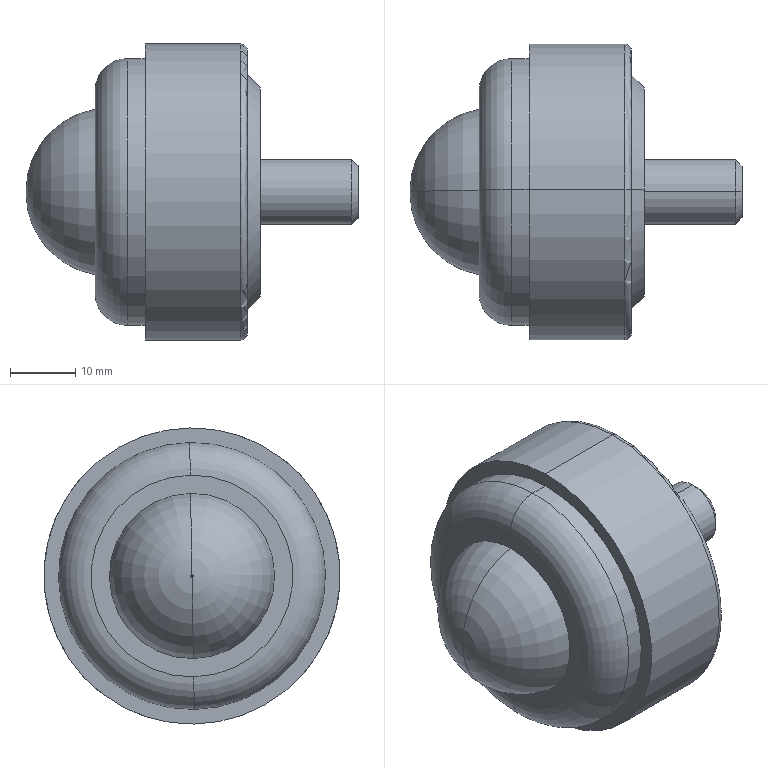Component | SolidWorks | GuideWheelAssembly-1_WD-03UniversalBall-1 | 1 solid | 22 faces | box 51 x 45.5 x 45.5 mm | volume 41338 mm3 | cylinder 6 | torus 6 | plane 6 | cone 4 | commonest cylinder face diameters 10 x2 41 x2 45.5 x2 | material Nylon 101
STEP:
#1=COLOUR_RGB('',0.7922,0.8196,0.9333);
#2=FILL_AREA_STYLE_COLOUR('',#1);
#3=FILL_AREA_STYLE('',(#2));
#4=SURFACE_STYLE_FILL_AREA(#3);
#5=SURFACE_SIDE_STYLE('',(#4));
#6=SURFACE_STYLE_USAGE(.BOTH.,#5);
#7=PRESENTATION_STYLE_ASSIGNMENT((#6));
#8=CARTESIAN_POINT('',(-21.614,-0.002693,0.8268));
#9=VERTEX_POINT('',#8);
#10=CARTESIAN_POINT('',(-21.614,0.002693,1.142));
#11=VERTEX_POINT('',#10);
#12=CARTESIAN_POINT('',(-21.614,-0.,0.9843));
#13=DIRECTION('',(1.,-0.,-0.));
#14=DIRECTION('',(0.,-0.0171,-0.9999));
#15=AXIS2_PLACEMENT_3D('',#12,#13,#14);
#16=CIRCLE('',#15,0.1575);
#17=EDGE_CURVE('',#9,#11,#16,.T.);
#18=ORIENTED_EDGE('',*,*,#17,.F.);
#19=CARTESIAN_POINT('',(-21.654,-0.003366,0.7874));
#20=VERTEX_POINT('',#19);
#21=CARTESIAN_POINT('',(-21.614,-0.002693,0.8268));
#22=DIRECTION('',(-0.7071,-0.01209,-0.707));
#23=VECTOR('',#22,39.37);
#24=LINE('',#21,#23);
#25=EDGE_CURVE('',#9,#20,#24,.T.);
#26=ORIENTED_EDGE('',*,*,#25,.T.);
#27=CARTESIAN_POINT('',(-21.654,0.003366,1.181));
#28=VERTEX_POINT('',#27);
#29=CARTESIAN_POINT('',(-21.654,-0.,0.9843));
#30=DIRECTION('',(-1.,0.,0.));
#31=DIRECTION('',(0.,-0.0171,-0.9999));
#32=AXIS2_PLACEMENT_3D('',#29,#30,#31);
#33=CIRCLE('',#32,0.1969);
#34=EDGE_CURVE('',#28,#20,#33,.T.);
#35=ORIENTED_EDGE('',*,*,#34,.F.);
#36=CARTESIAN_POINT('',(-21.614,0.002693,1.142));
#37=DIRECTION('',(-0.7071,0.01209,0.707));
#38=VECTOR('',#37,39.37);
#39=LINE('',#36,#38);
#40=EDGE_CURVE('',#11,#28,#39,.T.);
#41=ORIENTED_EDGE('',*,*,#40,.F.);
#42=EDGE_LOOP('',(#18,#26,#35,#41));
#43=FACE_OUTER_BOUND('',#42,.T.);
#44=CARTESIAN_POINT('',(-21.614,-0.,0.9843));
#45=DIRECTION('',(-1.,0.,0.));
#46=DIRECTION('',(0.,0.0171,0.9999));
#47=AXIS2_PLACEMENT_3D('',#44,#45,#46);
#48=CONICAL_SURFACE('',#47,0.1575,0.7854);
#49=ADVANCED_FACE('',(#43),#48,.T.);
#50=ORIENTED_EDGE('',*,*,#34,.T.);
#51=CARTESIAN_POINT('',(-22.205,-0.003366,0.7874));
#52=VERTEX_POINT('',#51);
#53=CARTESIAN_POINT('',(-21.614,-0.003366,0.7874));
#54=DIRECTION('',(-1.,0.,0.));
#55=VECTOR('',#54,39.37);
#56=LINE('',#53,#55);
#57=EDGE_CURVE('',#20,#52,#56,.T.);
#58=ORIENTED_EDGE('',*,*,#57,.T.);
#59=CARTESIAN_POINT('',(-22.205,0.003366,1.181));
#60=VERTEX_POINT('',#59);
#61=CARTESIAN_POINT('',(-22.205,-0.,0.9843));
#62=DIRECTION('',(1.,-0.,-0.));
#63=DIRECTION('',(0.,0.0171,0.9999));
#64=AXIS2_PLACEMENT_3D('',#61,#62,#63);
#65=CIRCLE('',#64,0.1969);
#66=EDGE_CURVE('',#52,#60,#65,.T.);
#67=ORIENTED_EDGE('',*,*,#66,.T.);
#68=CARTESIAN_POINT('',(-21.614,0.003366,1.181));
#69=DIRECTION('',(-1.,0.,0.));
#70=VECTOR('',#69,39.37);
#71=LINE('',#68,#70);
#72=EDGE_CURVE('',#28,#60,#71,.T.);
#73=ORIENTED_EDGE('',*,*,#72,.F.);
#74=EDGE_LOOP('',(#50,#58,#67,#73));
#75=FACE_OUTER_BOUND('',#74,.T.);
#76=CARTESIAN_POINT('',(-21.614,-0.,0.9843));
#77=DIRECTION('',(-1.,0.,0.));
#78=DIRECTION('',(0.,0.0171,0.9999));
#79=AXIS2_PLACEMENT_3D('',#76,#77,#78);
#80=CYLINDRICAL_SURFACE('',#79,0.1969);
#81=ADVANCED_FACE('',(#75),#80,.T.);
#82=CARTESIAN_POINT('',(-22.283,-0.01464,0.1281));
#83=VERTEX_POINT('',#82);
#84=CARTESIAN_POINT('',(-22.283,0.01464,1.84));
#85=VERTEX_POINT('',#84);
#86=CARTESIAN_POINT('',(-22.283,-0.,0.9843));
#87=DIRECTION('',(1.,-0.,-0.));
#88=DIRECTION('',(0.,0.0171,0.9999));
#89=AXIS2_PLACEMENT_3D('',#86,#87,#88);
#90=CIRCLE('',#89,0.8563);
#91=EDGE_CURVE('',#83,#85,#90,.T.);
#92=ORIENTED_EDGE('',*,*,#91,.F.);
#93=CARTESIAN_POINT('',(-22.323,-0.01532,0.08871));
#94=VERTEX_POINT('',#93);
#95=CARTESIAN_POINT('',(-22.323,-0.01464,0.1281));
#96=DIRECTION('',(0.,0.9999,-0.0171));
#97=DIRECTION('',(0.,0.0171,0.9999));
#98=AXIS2_PLACEMENT_3D('',#95,#96,#97);
#99=CIRCLE('',#98,0.03937);
#100=EDGE_CURVE('',#83,#94,#99,.T.);
#101=ORIENTED_EDGE('',*,*,#100,.T.);
#102=CARTESIAN_POINT('',(-22.323,0.01532,1.88));
#103=VERTEX_POINT('',#102);
#104=CARTESIAN_POINT('',(-22.323,-0.,0.9843));
#105=DIRECTION('',(-1.,0.,0.));
#106=DIRECTION('',(0.,0.0171,0.9999));
#107=AXIS2_PLACEMENT_3D('',#104,#105,#106);
#108=CIRCLE('',#107,0.8957);
#109=EDGE_CURVE('',#103,#94,#108,.T.);
#110=ORIENTED_EDGE('',*,*,#109,.F.);
#111=CARTESIAN_POINT('',(-22.323,0.01464,1.84));
#112=DIRECTION('',(-0.,-0.9999,0.0171));
#113=DIRECTION('',(0.,-0.0171,-0.9999));
#114=AXIS2_PLACEMENT_3D('',#111,#112,#113);
#115=CIRCLE('',#114,0.03937);
#116=EDGE_CURVE('',#85,#103,#115,.T.);
#117=ORIENTED_EDGE('',*,*,#116,.F.);
#118=EDGE_LOOP('',(#92,#101,#110,#117));
#119=FACE_OUTER_BOUND('',#118,.T.);
#120=CARTESIAN_POINT('',(-22.323,-0.,0.9843));
#121=DIRECTION('',(-1.,0.,0.));
#122=DIRECTION('',(0.,0.0171,0.9999));
#123=AXIS2_PLACEMENT_3D('',#120,#121,#122);
#124=TOROIDAL_SURFACE('',#123,0.8563,0.03937);
#125=ADVANCED_FACE('',(#119),#124,.T.);
#126=CARTESIAN_POINT('',(-22.205,-0.01077,0.3544));
#127=VERTEX_POINT('',#126);
#128=CARTESIAN_POINT('',(-22.205,0.01077,1.614));
#129=VERTEX_POINT('',#128);
#130=CARTESIAN_POINT('',(-22.205,-0.,0.9843));
#131=DIRECTION('',(1.,-0.,-0.));
#132=DIRECTION('',(0.,-0.0171,-0.9999));
#133=AXIS2_PLACEMENT_3D('',#130,#131,#132);
#134=CIRCLE('',#133,0.6299);
#135=EDGE_CURVE('',#127,#129,#134,.T.);
#136=ORIENTED_EDGE('',*,*,#135,.F.);
#137=CARTESIAN_POINT('',(-22.283,-0.01212,0.2757));
#138=VERTEX_POINT('',#137);
#139=CARTESIAN_POINT('',(-22.283,-0.01212,0.2757));
#140=DIRECTION('',(-0.7071,-0.01209,-0.707));
#141=VECTOR('',#140,39.37);
#142=LINE('',#139,#141);
#143=EDGE_CURVE('',#127,#138,#142,.T.);
#144=ORIENTED_EDGE('',*,*,#143,.T.);
#145=CARTESIAN_POINT('',(-22.283,0.01212,1.693));
#146=VERTEX_POINT('',#145);
#147=CARTESIAN_POINT('',(-22.283,-0.,0.9843));
#148=DIRECTION('',(1.,-0.,-0.));
#149=DIRECTION('',(0.,-0.0171,-0.9999));
#150=AXIS2_PLACEMENT_3D('',#147,#148,#149);
#151=CIRCLE('',#150,0.7087);
#152=EDGE_CURVE('',#138,#146,#151,.T.);
#153=ORIENTED_EDGE('',*,*,#152,.T.);
#154=CARTESIAN_POINT('',(-22.283,0.01212,1.693));
#155=DIRECTION('',(-0.7071,0.01209,0.707));
#156=VECTOR('',#155,39.37);
#157=LINE('',#154,#156);
#158=EDGE_CURVE('',#129,#146,#157,.T.);
#159=ORIENTED_EDGE('',*,*,#158,.F.);
#160=EDGE_LOOP('',(#136,#144,#153,#159));
#161=FACE_OUTER_BOUND('',#160,.T.);
#162=CARTESIAN_POINT('',(-22.283,-0.,0.9843));
#163=DIRECTION('',(-1.,0.,0.));
#164=DIRECTION('',(0.,0.0171,0.9999));
#165=AXIS2_PLACEMENT_3D('',#162,#163,#164);
#166=CONICAL_SURFACE('',#165,0.7087,0.7854);
#167=ADVANCED_FACE('',(#161),#166,.T.);
#168=CARTESIAN_POINT('',(-23.008,-0.0138,0.1773));
#169=VERTEX_POINT('',#168);
#170=CARTESIAN_POINT('',(-23.008,0.0138,1.791));
#171=VERTEX_POINT('',#170);
#172=CARTESIAN_POINT('',(-23.008,-0.,0.9843));
#173=DIRECTION('',(1.,-0.,-0.));
#174=DIRECTION('',(0.,0.0171,0.9999));
#175=AXIS2_PLACEMENT_3D('',#172,#173,#174);
#176=CIRCLE('',#175,0.8071);
#177=EDGE_CURVE('',#169,#171,#176,.T.);
#178=ORIENTED_EDGE('',*,*,#177,.F.);
#179=CARTESIAN_POINT('',(-23.205,-0.01044,0.3741));
#180=VERTEX_POINT('',#179);
#181=CARTESIAN_POINT('',(-23.008,-0.01044,0.3741));
#182=DIRECTION('',(0.,0.9999,-0.0171));
#183=DIRECTION('',(0.,0.0171,0.9999));
#184=AXIS2_PLACEMENT_3D('',#181,#182,#183);
#185=CIRCLE('',#184,0.1969);
#186=EDGE_CURVE('',#169,#180,#185,.T.);
#187=ORIENTED_EDGE('',*,*,#186,.T.);
#188=CARTESIAN_POINT('',(-23.205,0.01044,1.594));
#189=VERTEX_POINT('',#188);
#190=CARTESIAN_POINT('',(-23.205,-0.,0.9843));
#191=DIRECTION('',(-1.,0.,0.));
#192=DIRECTION('',(0.,0.0171,0.9999));
#193=AXIS2_PLACEMENT_3D('',#190,#191,#192);
#194=CIRCLE('',#193,0.6102);
#195=EDGE_CURVE('',#189,#180,#194,.T.);
#196=ORIENTED_EDGE('',*,*,#195,.F.);
#197=CARTESIAN_POINT('',(-23.008,0.01044,1.594));
#198=DIRECTION('',(-0.,-0.9999,0.0171));
#199=DIRECTION('',(0.,-0.0171,-0.9999));
#200=AXIS2_PLACEMENT_3D('',#197,#198,#199);
#201=CIRCLE('',#200,0.1969);
#202=EDGE_CURVE('',#171,#189,#201,.T.);
#203=ORIENTED_EDGE('',*,*,#202,.F.);
#204=EDGE_LOOP('',(#178,#187,#196,#203));
#205=FACE_OUTER_BOUND('',#204,.T.);
#206=CARTESIAN_POINT('',(-23.008,-0.,0.9843));
#207=DIRECTION('',(-1.,0.,0.));
#208=DIRECTION('',(0.,0.0171,0.9999));
#209=AXIS2_PLACEMENT_3D('',#206,#207,#208);
#210=TOROIDAL_SURFACE('',#209,0.6102,0.1969);
#211=ADVANCED_FACE('',(#205),#210,.T.);
#212=CARTESIAN_POINT('',(-23.622,0.0001177,0.9911));
#213=VERTEX_POINT('',#212);
#214=CARTESIAN_POINT('',(-23.622,-0.0001177,0.9774));
#215=VERTEX_POINT('',#214);
#216=CARTESIAN_POINT('',(-23.622,-0.,0.9843));
#217=DIRECTION('',(-1.,0.,0.));
#218=DIRECTION('',(0.,0.0171,0.9999));
#219=AXIS2_PLACEMENT_3D('',#216,#217,#218);
#220=CIRCLE('',#219,0.006883);
#221=EDGE_CURVE('',#213,#215,#220,.T.);
#222=ORIENTED_EDGE('',*,*,#221,.F.);
#223=CARTESIAN_POINT('',(-23.205,0.00855,1.484));
#224=VERTEX_POINT('',#223);
#225=CARTESIAN_POINT('',(-23.122,0.0001177,0.9911));
#226=DIRECTION('',(0.,0.9999,-0.0171));
#227=DIRECTION('',(0.,0.0171,0.9999));
#228=AXIS2_PLACEMENT_3D('',#225,#226,#227);
#229=CIRCLE('',#228,0.5);
#230=EDGE_CURVE('',#213,#224,#229,.T.);
#231=ORIENTED_EDGE('',*,*,#230,.T.);
#232=CARTESIAN_POINT('',(-23.205,-0.00855,0.4843));
#233=VERTEX_POINT('',#232);
#234=CARTESIAN_POINT('',(-23.205,-0.,0.9843));
#235=DIRECTION('',(1.,-0.,-0.));
#236=DIRECTION('',(0.,0.0171,0.9999));
#237=AXIS2_PLACEMENT_3D('',#234,#235,#236);
#238=CIRCLE('',#237,0.5);
#239=EDGE_CURVE('',#233,#224,#238,.T.);
#240=ORIENTED_EDGE('',*,*,#239,.F.);
#241=CARTESIAN_POINT('',(-23.122,-0.0001177,0.9774));
#242=DIRECTION('',(-0.,-0.9999,0.0171));
#243=DIRECTION('',(0.,-0.0171,-0.9999));
#244=AXIS2_PLACEMENT_3D('',#241,#242,#243);
#245=CIRCLE('',#244,0.5);
#246=EDGE_CURVE('',#215,#233,#245,.T.);
#247=ORIENTED_EDGE('',*,*,#246,.F.);
#248=EDGE_LOOP('',(#222,#231,#240,#247));
#249=FACE_OUTER_BOUND('',#248,.T.);
#250=CARTESIAN_POINT('',(-23.122,-0.,0.9843));
#251=DIRECTION('',(1.,-0.,-0.));
#252=DIRECTION('',(-0.,-0.0171,-0.9999));
#253=AXIS2_PLACEMENT_3D('',#250,#251,#252);
#254=TOROIDAL_SURFACE('',#253,0.006883,0.5);
#255=ADVANCED_FACE('',(#249),#254,.T.);
#256=ORIENTED_EDGE('',*,*,#177,.T.);
#257=CARTESIAN_POINT('',(-22.902,0.0138,1.791));
#258=VERTEX_POINT('',#257);
#259=CARTESIAN_POINT('',(-23.205,0.0138,1.791));
#260=DIRECTION('',(1.,-0.,-0.));
#261=VECTOR('',#260,39.37);
#262=LINE('',#259,#261);
#263=EDGE_CURVE('',#171,#258,#262,.T.);
#264=ORIENTED_EDGE('',*,*,#263,.T.);
#265=CARTESIAN_POINT('',(-22.902,-0.0138,0.1773));
#266=VERTEX_POINT('',#265);
#267=CARTESIAN_POINT('',(-22.902,-0.,0.9843));
#268=DIRECTION('',(-1.,0.,0.));
#269=DIRECTION('',(0.,0.0171,0.9999));
#270=AXIS2_PLACEMENT_3D('',#267,#268,#269);
#271=CIRCLE('',#270,0.8071);
#272=EDGE_CURVE('',#258,#266,#271,.T.);
#273=ORIENTED_EDGE('',*,*,#272,.T.);
#274=CARTESIAN_POINT('',(-23.205,-0.0138,0.1773));
#275=DIRECTION('',(1.,-0.,-0.));
#276=VECTOR('',#275,39.37);
#277=LINE('',#274,#276);
#278=EDGE_CURVE('',#169,#266,#277,.T.);
#279=ORIENTED_EDGE('',*,*,#278,.F.);
#280=EDGE_LOOP('',(#256,#264,#273,#279));
#281=FACE_OUTER_BOUND('',#280,.T.);
#282=CARTESIAN_POINT('',(-23.205,-0.,0.9843));
#283=DIRECTION('',(1.,-0.,-0.));
#284=DIRECTION('',(0.,-0.0171,-0.9999));
#285=AXIS2_PLACEMENT_3D('',#282,#283,#284);
#286=CYLINDRICAL_SURFACE('',#285,0.8071);
#287=ADVANCED_FACE('',(#281),#286,.T.);
#288=CARTESIAN_POINT('',(-22.902,0.01532,1.88));
#289=VERTEX_POINT('',#288);
#290=CARTESIAN_POINT('',(-22.902,-0.01532,0.08871));
#291=VERTEX_POINT('',#290);
#292=CARTESIAN_POINT('',(-22.902,-0.,0.9843));
#293=DIRECTION('',(-1.,0.,0.));
#294=DIRECTION('',(0.,0.0171,0.9999));
#295=AXIS2_PLACEMENT_3D('',#292,#293,#294);
#296=CIRCLE('',#295,0.8957);
#297=EDGE_CURVE('',#289,#291,#296,.T.);
#298=ORIENTED_EDGE('',*,*,#297,.F.);
#299=CARTESIAN_POINT('',(-22.902,0.01532,1.88));
#300=DIRECTION('',(1.,-0.,-0.));
#301=VECTOR('',#300,39.37);
#302=LINE('',#299,#301);
#303=EDGE_CURVE('',#289,#103,#302,.T.);
#304=ORIENTED_EDGE('',*,*,#303,.T.);
#305=ORIENTED_EDGE('',*,*,#109,.T.);
#306=CARTESIAN_POINT('',(-22.902,-0.01532,0.08871));
#307=DIRECTION('',(1.,-0.,-0.));
#308=VECTOR('',#307,39.37);
#309=LINE('',#306,#308);
#310=EDGE_CURVE('',#291,#94,#309,.T.);
#311=ORIENTED_EDGE('',*,*,#310,.F.);
#312=EDGE_LOOP('',(#298,#304,#305,#311));
#313=FACE_OUTER_BOUND('',#312,.T.);
#314=CARTESIAN_POINT('',(-22.902,-0.,0.9843));
#315=DIRECTION('',(1.,-0.,-0.));
#316=DIRECTION('',(0.,-0.0171,-0.9999));
#317=AXIS2_PLACEMENT_3D('',#314,#315,#316);
#318=CYLINDRICAL_SURFACE('',#317,0.8957);
#319=ADVANCED_FACE('',(#313),#318,.T.);
#320=CARTESIAN_POINT('',(-22.205,-0.,0.9843));
#321=DIRECTION('',(1.,-0.,-0.));
#322=DIRECTION('',(0.,-0.0171,-0.9999));
#323=AXIS2_PLACEMENT_3D('',#320,#321,#322);
#324=CIRCLE('',#323,0.6299);
#325=EDGE_CURVE('',#129,#127,#324,.T.);
#326=ORIENTED_EDGE('',*,*,#325,.T.);
#327=ORIENTED_EDGE('',*,*,#135,.T.);
#328=EDGE_LOOP('',(#326,#327));
#329=FACE_OUTER_BOUND('',#328,.T.);
#330=CARTESIAN_POINT('',(-22.205,-0.,0.9843));
#331=DIRECTION('',(1.,-0.,-0.));
#332=DIRECTION('',(0.,0.0171,0.9999));
#333=AXIS2_PLACEMENT_3D('',#330,#331,#332);
#334=CIRCLE('',#333,0.1969);
#335=EDGE_CURVE('',#60,#52,#334,.T.);
#336=ORIENTED_EDGE('',*,*,#335,.F.);
#337=ORIENTED_EDGE('',*,*,#66,.F.);
#338=EDGE_LOOP('',(#336,#337));
#339=FACE_BOUND('',#338,.T.);
#340=CARTESIAN_POINT('',(-22.205,-0.,0.9843));
#341=DIRECTION('',(-1.,0.,0.));
#342=DIRECTION('',(0.,0.0171,0.9999));
#343=AXIS2_PLACEMENT_3D('',#340,#341,#342);
#344=PLANE('',#343);
#345=ADVANCED_FACE('',(#329,#339),#344,.F.);
#346=ORIENTED_EDGE('',*,*,#195,.T.);
#347=CARTESIAN_POINT('',(-23.205,-0.,0.9843));
#348=DIRECTION('',(-1.,0.,0.));
#349=DIRECTION('',(0.,0.0171,0.9999));
#350=AXIS2_PLACEMENT_3D('',#347,#348,#349);
#351=CIRCLE('',#350,0.6102);
#352=EDGE_CURVE('',#180,#189,#351,.T.);
#353=ORIENTED_EDGE('',*,*,#352,.T.);
#354=EDGE_LOOP('',(#346,#353));
#355=FACE_OUTER_BOUND('',#354,.T.);
#356=ORIENTED_EDGE('',*,*,#239,.T.);
#357=CARTESIAN_POINT('',(-23.205,-0.,0.9843));
#358=DIRECTION('',(1.,-0.,-0.));
#359=DIRECTION('',(0.,0.0171,0.9999));
#360=AXIS2_PLACEMENT_3D('',#357,#358,#359);
#361=CIRCLE('',#360,0.5);
#362=EDGE_CURVE('',#224,#233,#361,.T.);
#363=ORIENTED_EDGE('',*,*,#362,.T.);
#364=EDGE_LOOP('',(#356,#363));
#365=FACE_BOUND('',#364,.T.);
#366=CARTESIAN_POINT('',(-23.205,-0.,0.9843));
#367=DIRECTION('',(-1.,0.,0.));
#368=DIRECTION('',(0.,0.0171,0.9999));
#369=AXIS2_PLACEMENT_3D('',#366,#367,#368);
#370=PLANE('',#369);
#371=ADVANCED_FACE('',(#355,#365),#370,.T.);
#372=CARTESIAN_POINT('',(-22.902,-0.,0.9843));
#373=DIRECTION('',(-1.,0.,0.));
#374=DIRECTION('',(0.,0.0171,0.9999));
#375=AXIS2_PLACEMENT_3D('',#372,#373,#374);
#376=CIRCLE('',#375,0.8957);
#377=EDGE_CURVE('',#291,#289,#376,.T.);
#378=ORIENTED_EDGE('',*,*,#377,.T.);
#379=ORIENTED_EDGE('',*,*,#297,.T.);
#380=EDGE_LOOP('',(#378,#379));
#381=FACE_OUTER_BOUND('',#380,.T.);
#382=CARTESIAN_POINT('',(-22.902,-0.,0.9843));
#383=DIRECTION('',(-1.,0.,0.));
#384=DIRECTION('',(0.,0.0171,0.9999));
#385=AXIS2_PLACEMENT_3D('',#382,#383,#384);
#386=CIRCLE('',#385,0.8071);
#387=EDGE_CURVE('',#266,#258,#386,.T.);
#388=ORIENTED_EDGE('',*,*,#387,.F.);
#389=ORIENTED_EDGE('',*,*,#272,.F.);
#390=EDGE_LOOP('',(#388,#389));
#391=FACE_BOUND('',#390,.T.);
#392=CARTESIAN_POINT('',(-22.902,-0.,0.9843));
#393=DIRECTION('',(-1.,0.,0.));
#394=DIRECTION('',(0.,0.0171,0.9999));
#395=AXIS2_PLACEMENT_3D('',#392,#393,#394);
#396=PLANE('',#395);
#397=ADVANCED_FACE('',(#381,#391),#396,.T.);
#398=ORIENTED_EDGE('',*,*,#303,.F.);
#399=ORIENTED_EDGE('',*,*,#377,.F.);
#400=ORIENTED_EDGE('',*,*,#310,.T.);
#401=CARTESIAN_POINT('',(-22.323,-0.,0.9843));
#402=DIRECTION('',(-1.,0.,0.));
#403=DIRECTION('',(0.,0.0171,0.9999));
#404=AXIS2_PLACEMENT_3D('',#401,#402,#403);
#405=CIRCLE('',#404,0.8957);
#406=EDGE_CURVE('',#94,#103,#405,.T.);
#407=ORIENTED_EDGE('',*,*,#406,.T.);
#408=EDGE_LOOP('',(#398,#399,#400,#407));
#409=FACE_OUTER_BOUND('',#408,.T.);
#410=CARTESIAN_POINT('',(-22.902,-0.,0.9843));
#411=DIRECTION('',(1.,-0.,-0.));
#412=DIRECTION('',(0.,-0.0171,-0.9999));
#413=AXIS2_PLACEMENT_3D('',#410,#411,#412);
#414=CYLINDRICAL_SURFACE('',#413,0.8957);
#415=ADVANCED_FACE('',(#409),#414,.T.);
#416=ORIENTED_EDGE('',*,*,#263,.F.);
#417=CARTESIAN_POINT('',(-23.008,-0.,0.9843));
#418=DIRECTION('',(1.,-0.,-0.));
#419=DIRECTION('',(0.,0.0171,0.9999));
#420=AXIS2_PLACEMENT_3D('',#417,#418,#419);
#421=CIRCLE('',#420,0.8071);
#422=EDGE_CURVE('',#171,#169,#421,.T.);
#423=ORIENTED_EDGE('',*,*,#422,.T.);
#424=ORIENTED_EDGE('',*,*,#278,.T.);
#425=ORIENTED_EDGE('',*,*,#387,.T.);
#426=EDGE_LOOP('',(#416,#423,#424,#425));
#427=FACE_OUTER_BOUND('',#426,.T.);
#428=CARTESIAN_POINT('',(-23.205,-0.,0.9843));
#429=DIRECTION('',(1.,-0.,-0.));
#430=DIRECTION('',(0.,-0.0171,-0.9999));
#431=AXIS2_PLACEMENT_3D('',#428,#429,#430);
#432=CYLINDRICAL_SURFACE('',#431,0.8071);
#433=ADVANCED_FACE('',(#427),#432,.T.);
#434=CARTESIAN_POINT('',(-23.622,-0.,0.9843));
#435=DIRECTION('',(-1.,0.,0.));
#436=DIRECTION('',(0.,0.0171,0.9999));
#437=AXIS2_PLACEMENT_3D('',#434,#435,#436);
#438=CIRCLE('',#437,0.006883);
#439=EDGE_CURVE('',#215,#213,#438,.T.);
#440=ORIENTED_EDGE('',*,*,#439,.T.);
#441=ORIENTED_EDGE('',*,*,#221,.T.);
#442=EDGE_LOOP('',(#440,#441));
#443=FACE_OUTER_BOUND('',#442,.T.);
#444=CARTESIAN_POINT('',(-23.622,-0.,0.9843));
#445=DIRECTION('',(-1.,0.,0.));
#446=DIRECTION('',(0.,0.0171,0.9999));
#447=AXIS2_PLACEMENT_3D('',#444,#445,#446);
#448=PLANE('',#447);
#449=ADVANCED_FACE('',(#443),#448,.T.);
#450=ORIENTED_EDGE('',*,*,#230,.F.);
#451=ORIENTED_EDGE('',*,*,#439,.F.);
#452=ORIENTED_EDGE('',*,*,#246,.T.);
#453=ORIENTED_EDGE('',*,*,#362,.F.);
#454=EDGE_LOOP('',(#450,#451,#452,#453));
#455=FACE_OUTER_BOUND('',#454,.T.);
#456=CARTESIAN_POINT('',(-23.122,-0.,0.9843));
#457=DIRECTION('',(1.,-0.,-0.));
#458=DIRECTION('',(-0.,-0.0171,-0.9999));
#459=AXIS2_PLACEMENT_3D('',#456,#457,#458);
#460=TOROIDAL_SURFACE('',#459,0.006883,0.5);
#461=ADVANCED_FACE('',(#455),#460,.T.);
#462=ORIENTED_EDGE('',*,*,#186,.F.);
#463=ORIENTED_EDGE('',*,*,#422,.F.);
#464=ORIENTED_EDGE('',*,*,#202,.T.);
#465=ORIENTED_EDGE('',*,*,#352,.F.);
#466=EDGE_LOOP('',(#462,#463,#464,#465));
#467=FACE_OUTER_BOUND('',#466,.T.);
#468=CARTESIAN_POINT('',(-23.008,-0.,0.9843));
#469=DIRECTION('',(-1.,0.,0.));
#470=DIRECTION('',(0.,0.0171,0.9999));
#471=AXIS2_PLACEMENT_3D('',#468,#469,#470);
#472=TOROIDAL_SURFACE('',#471,0.6102,0.1969);
#473=ADVANCED_FACE('',(#467),#472,.T.);
#474=CARTESIAN_POINT('',(-22.283,-0.,0.9843));
#475=DIRECTION('',(1.,-0.,-0.));
#476=DIRECTION('',(0.,0.0171,0.9999));
#477=AXIS2_PLACEMENT_3D('',#474,#475,#476);
#478=CIRCLE('',#477,0.8563);
#479=EDGE_CURVE('',#85,#83,#478,.T.);
#480=ORIENTED_EDGE('',*,*,#479,.T.);
#481=ORIENTED_EDGE('',*,*,#91,.T.);
#482=EDGE_LOOP('',(#480,#481));
#483=FACE_OUTER_BOUND('',#482,.T.);
#484=CARTESIAN_POINT('',(-22.283,-0.,0.9843));
#485=DIRECTION('',(1.,-0.,-0.));
#486=DIRECTION('',(0.,-0.0171,-0.9999));
#487=AXIS2_PLACEMENT_3D('',#484,#485,#486);
#488=CIRCLE('',#487,0.7087);
#489=EDGE_CURVE('',#146,#138,#488,.T.);
#490=ORIENTED_EDGE('',*,*,#489,.F.);
#491=ORIENTED_EDGE('',*,*,#152,.F.);
#492=EDGE_LOOP('',(#490,#491));
#493=FACE_BOUND('',#492,.T.);
#494=CARTESIAN_POINT('',(-22.283,0.7086,0.9721));
#495=DIRECTION('',(-1.,0.,0.));
#496=DIRECTION('',(0.,0.0171,0.9999));
#497=AXIS2_PLACEMENT_3D('',#494,#495,#496);
#498=PLANE('',#497);
#499=ADVANCED_FACE('',(#483,#493),#498,.F.);
#500=ORIENTED_EDGE('',*,*,#143,.F.);
#501=ORIENTED_EDGE('',*,*,#325,.F.);
#502=ORIENTED_EDGE('',*,*,#158,.T.);
#503=ORIENTED_EDGE('',*,*,#489,.T.);
#504=EDGE_LOOP('',(#500,#501,#502,#503));
#505=FACE_OUTER_BOUND('',#504,.T.);
#506=CARTESIAN_POINT('',(-22.283,-0.,0.9843));
#507=DIRECTION('',(-1.,0.,0.));
#508=DIRECTION('',(0.,0.0171,0.9999));
#509=AXIS2_PLACEMENT_3D('',#506,#507,#508);
#510=CONICAL_SURFACE('',#509,0.7087,0.7854);
#511=ADVANCED_FACE('',(#505),#510,.T.);
#512=ORIENTED_EDGE('',*,*,#100,.F.);
#513=ORIENTED_EDGE('',*,*,#479,.F.);
#514=ORIENTED_EDGE('',*,*,#116,.T.);
#515=ORIENTED_EDGE('',*,*,#406,.F.);
#516=EDGE_LOOP('',(#512,#513,#514,#515));
#517=FACE_OUTER_BOUND('',#516,.T.);
#518=CARTESIAN_POINT('',(-22.323,-0.,0.9843));
#519=DIRECTION('',(-1.,0.,0.));
#520=DIRECTION('',(0.,0.0171,0.9999));
#521=AXIS2_PLACEMENT_3D('',#518,#519,#520);
#522=TOROIDAL_SURFACE('',#521,0.8563,0.03937);
#523=ADVANCED_FACE('',(#517),#522,.T.);
#524=ORIENTED_EDGE('',*,*,#57,.F.);
#525=CARTESIAN_POINT('',(-21.654,-0.,0.9843));
#526=DIRECTION('',(-1.,0.,0.));
#527=DIRECTION('',(0.,-0.0171,-0.9999));
#528=AXIS2_PLACEMENT_3D('',#525,#526,#527);
#529=CIRCLE('',#528,0.1969);
#530=EDGE_CURVE('',#20,#28,#529,.T.);
#531=ORIENTED_EDGE('',*,*,#530,.T.);
#532=ORIENTED_EDGE('',*,*,#72,.T.);
#533=ORIENTED_EDGE('',*,*,#335,.T.);
#534=EDGE_LOOP('',(#524,#531,#532,#533));
#535=FACE_OUTER_BOUND('',#534,.T.);
#536=CARTESIAN_POINT('',(-21.614,-0.,0.9843));
#537=DIRECTION('',(-1.,0.,0.));
#538=DIRECTION('',(0.,0.0171,0.9999));
#539=AXIS2_PLACEMENT_3D('',#536,#537,#538);
#540=CYLINDRICAL_SURFACE('',#539,0.1969);
#541=ADVANCED_FACE('',(#535),#540,.T.);
#542=CARTESIAN_POINT('',(-21.614,-0.,0.9843));
#543=DIRECTION('',(1.,-0.,-0.));
#544=DIRECTION('',(0.,-0.0171,-0.9999));
#545=AXIS2_PLACEMENT_3D('',#542,#543,#544);
#546=CIRCLE('',#545,0.1575);
#547=EDGE_CURVE('',#11,#9,#546,.T.);
#548=ORIENTED_EDGE('',*,*,#547,.T.);
#549=ORIENTED_EDGE('',*,*,#17,.T.);
#550=EDGE_LOOP('',(#548,#549));
#551=FACE_OUTER_BOUND('',#550,.T.);
#552=CARTESIAN_POINT('',(-21.614,-0.,0.9843));
#553=DIRECTION('',(1.,-0.,-0.));
#554=DIRECTION('',(-0.,-0.0171,-0.9999));
#555=AXIS2_PLACEMENT_3D('',#552,#553,#554);
#556=PLANE('',#555);
#557=ADVANCED_FACE('',(#551),#556,.T.);
#558=ORIENTED_EDGE('',*,*,#25,.F.);
#559=ORIENTED_EDGE('',*,*,#547,.F.);
#560=ORIENTED_EDGE('',*,*,#40,.T.);
#561=ORIENTED_EDGE('',*,*,#530,.F.);
#562=EDGE_LOOP('',(#558,#559,#560,#561));
#563=FACE_OUTER_BOUND('',#562,.T.);
#564=CARTESIAN_POINT('',(-21.614,-0.,0.9843));
#565=DIRECTION('',(-1.,0.,0.));
#566=DIRECTION('',(0.,0.0171,0.9999));
#567=AXIS2_PLACEMENT_3D('',#564,#565,#566);
#568=CONICAL_SURFACE('',#567,0.1575,0.7854);
#569=ADVANCED_FACE('',(#563),#568,.T.);
#570=CLOSED_SHELL('',(#49,#81,#125,#167,#211,#255,#287,#319,#345,#371,#397,#415,#433,#449,#461,#473,#499,#511,#523,#541,#557,#569));
#571=MANIFOLD_SOLID_BREP('',#570);
#572=STYLED_ITEM('',(#7),#571);
#573=PRESENTATION_LAYER_ASSIGNMENT('','',(#572));
#574=CARTESIAN_POINT('',(0.,0.,0.));
#575=DIRECTION('',(0.,0.,1.));
#576=DIRECTION('',(1.,0.,0.));
#577=AXIS2_PLACEMENT_3D('',#574,#575,#576);
#578=(LENGTH_UNIT()NAMED_UNIT(*)SI_UNIT($,.METRE.));
#579=LENGTH_MEASURE_WITH_UNIT(LENGTH_MEASURE(0.0254),#578);
#580=DIMENSIONAL_EXPONENTS(1.,0.,0.,0.,0.,0.,0.);
#581=(CONVERSION_BASED_UNIT('',#579)LENGTH_UNIT()NAMED_UNIT(#580));
#582=UNCERTAINTY_MEASURE_WITH_UNIT(LENGTH_MEASURE(0.00001),#581,'','');
#583=(NAMED_UNIT(*)PLANE_ANGLE_UNIT()SI_UNIT($,.RADIAN.));
#584=(NAMED_UNIT(*)SI_UNIT($,.STERADIAN.)SOLID_ANGLE_UNIT());
#585=(GEOMETRIC_REPRESENTATION_CONTEXT(3)GLOBAL_UNCERTAINTY_ASSIGNED_CONTEXT((#582))GLOBAL_UNIT_ASSIGNED_CONTEXT((#581,#583,#584))REPRESENTATION_CONTEXT('',''));
#586=ADVANCED_BREP_SHAPE_REPRESENTATION('',(#571,#577),#585);
#587=(LENGTH_UNIT()NAMED_UNIT(*)SI_UNIT($,.METRE.));
#588=LENGTH_MEASURE_WITH_UNIT(LENGTH_MEASURE(0.0254),#587);
#589=DIMENSIONAL_EXPONENTS(1.,0.,0.,0.,0.,0.,0.);
#590=(CONVERSION_BASED_UNIT('',#588)LENGTH_UNIT()NAMED_UNIT(#589));
#591=UNCERTAINTY_MEASURE_WITH_UNIT(LENGTH_MEASURE(0.00001),#590,'','');
#592=(NAMED_UNIT(*)PLANE_ANGLE_UNIT()SI_UNIT($,.RADIAN.));
#593=(NAMED_UNIT(*)SI_UNIT($,.STERADIAN.)SOLID_ANGLE_UNIT());
#594=(GEOMETRIC_REPRESENTATION_CONTEXT(3)GLOBAL_UNCERTAINTY_ASSIGNED_CONTEXT((#591))GLOBAL_UNIT_ASSIGNED_CONTEXT((#590,#592,#593))REPRESENTATION_CONTEXT('',''));
#595=MECHANICAL_DESIGN_GEOMETRIC_PRESENTATION_REPRESENTATION('',(#572),#594);